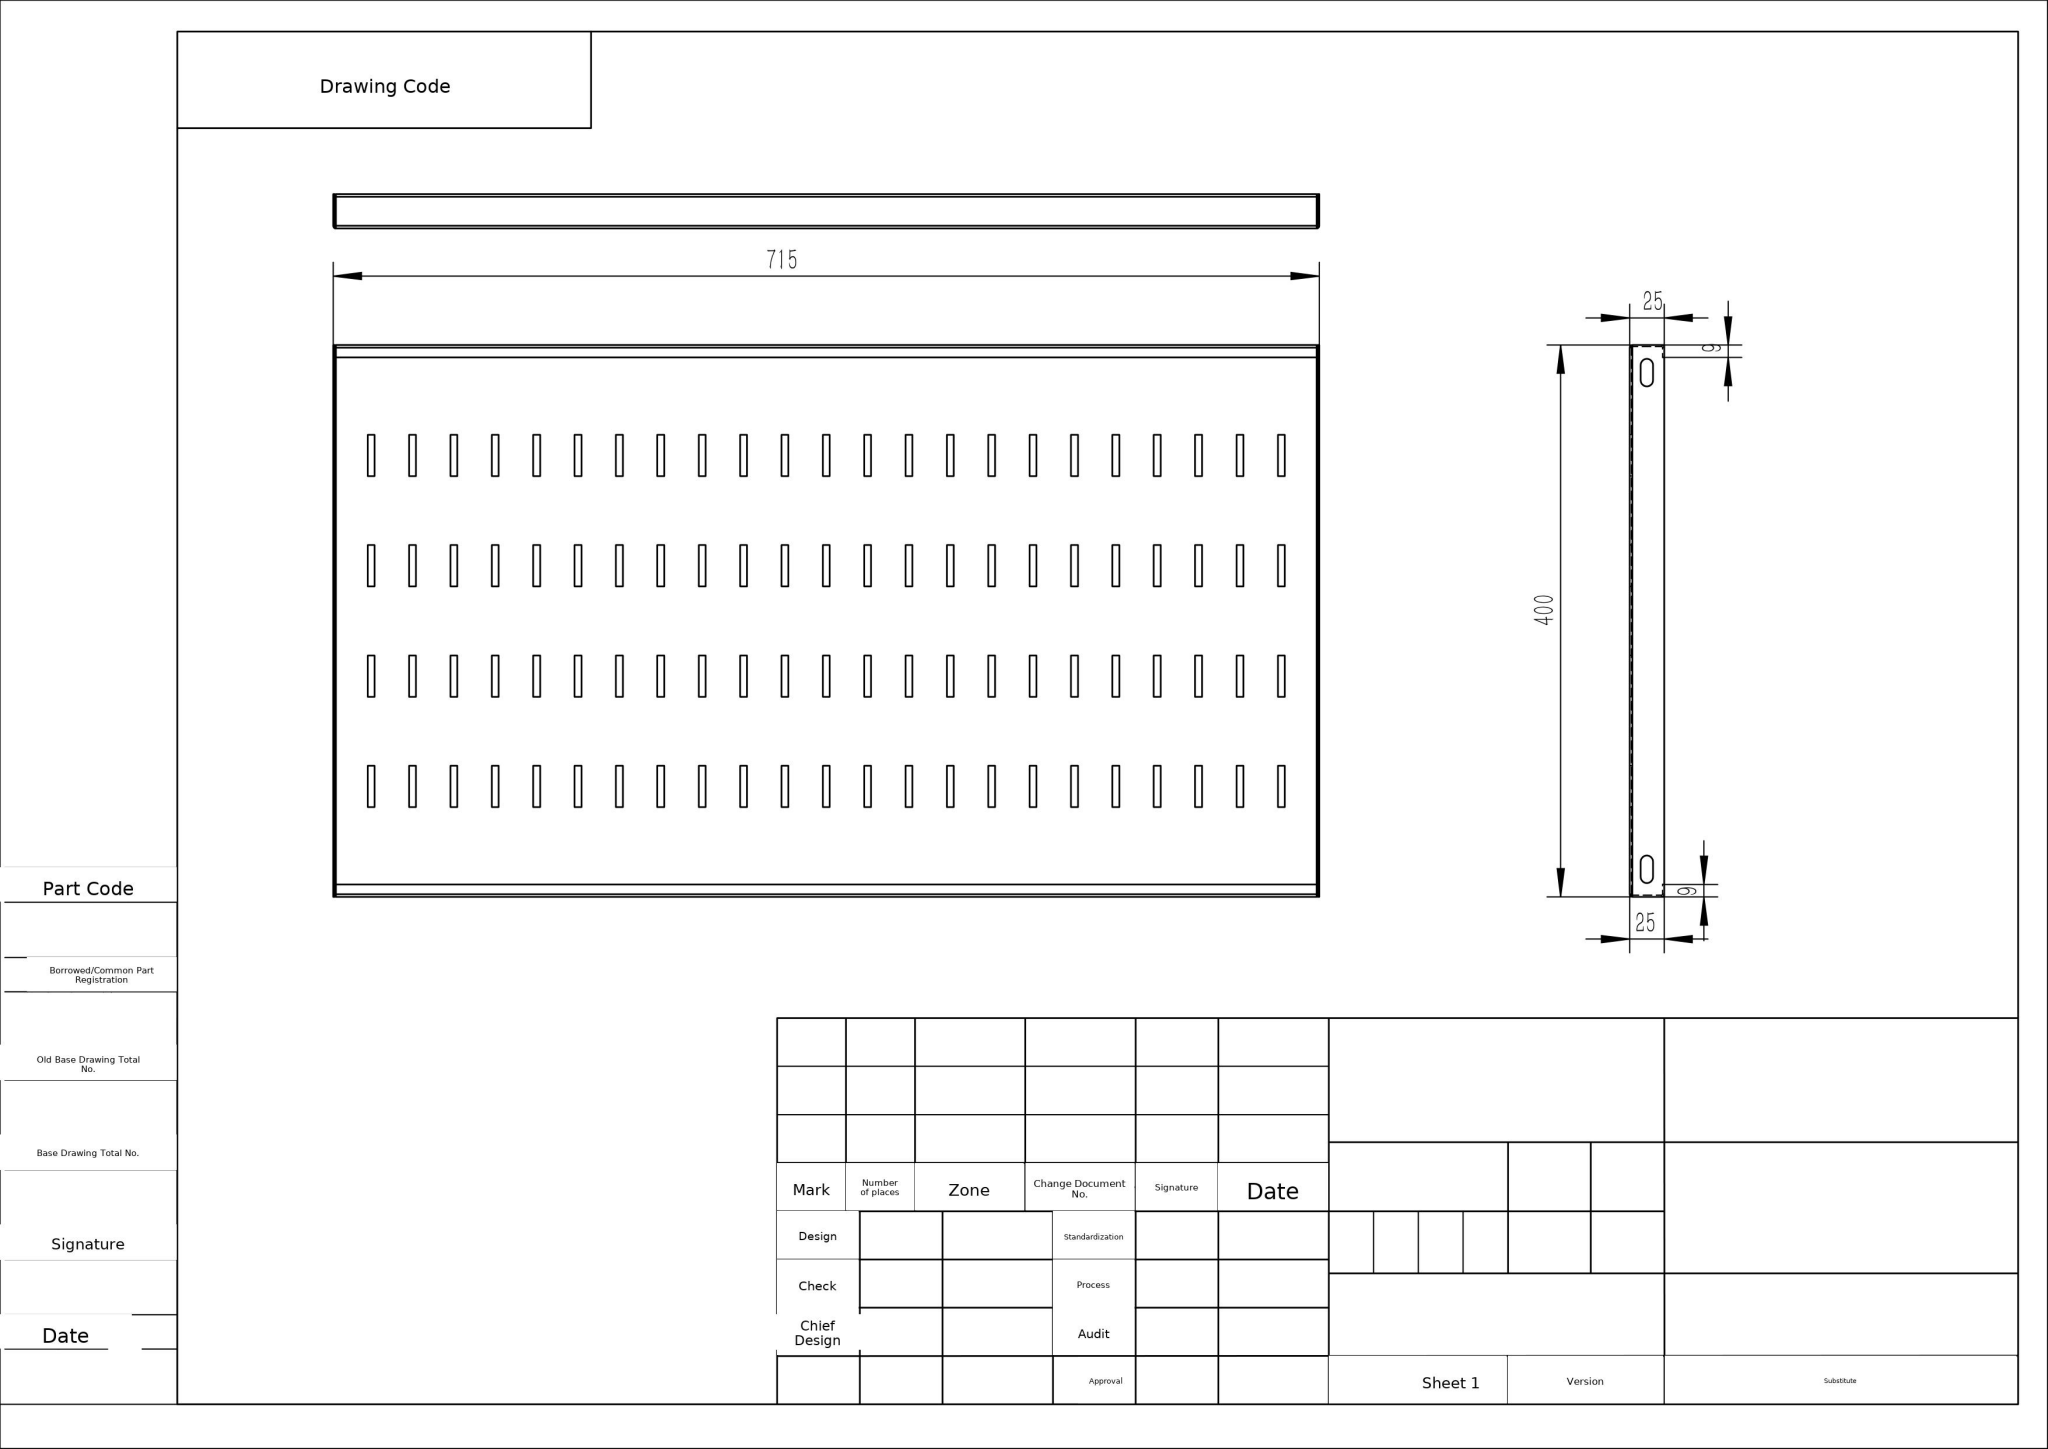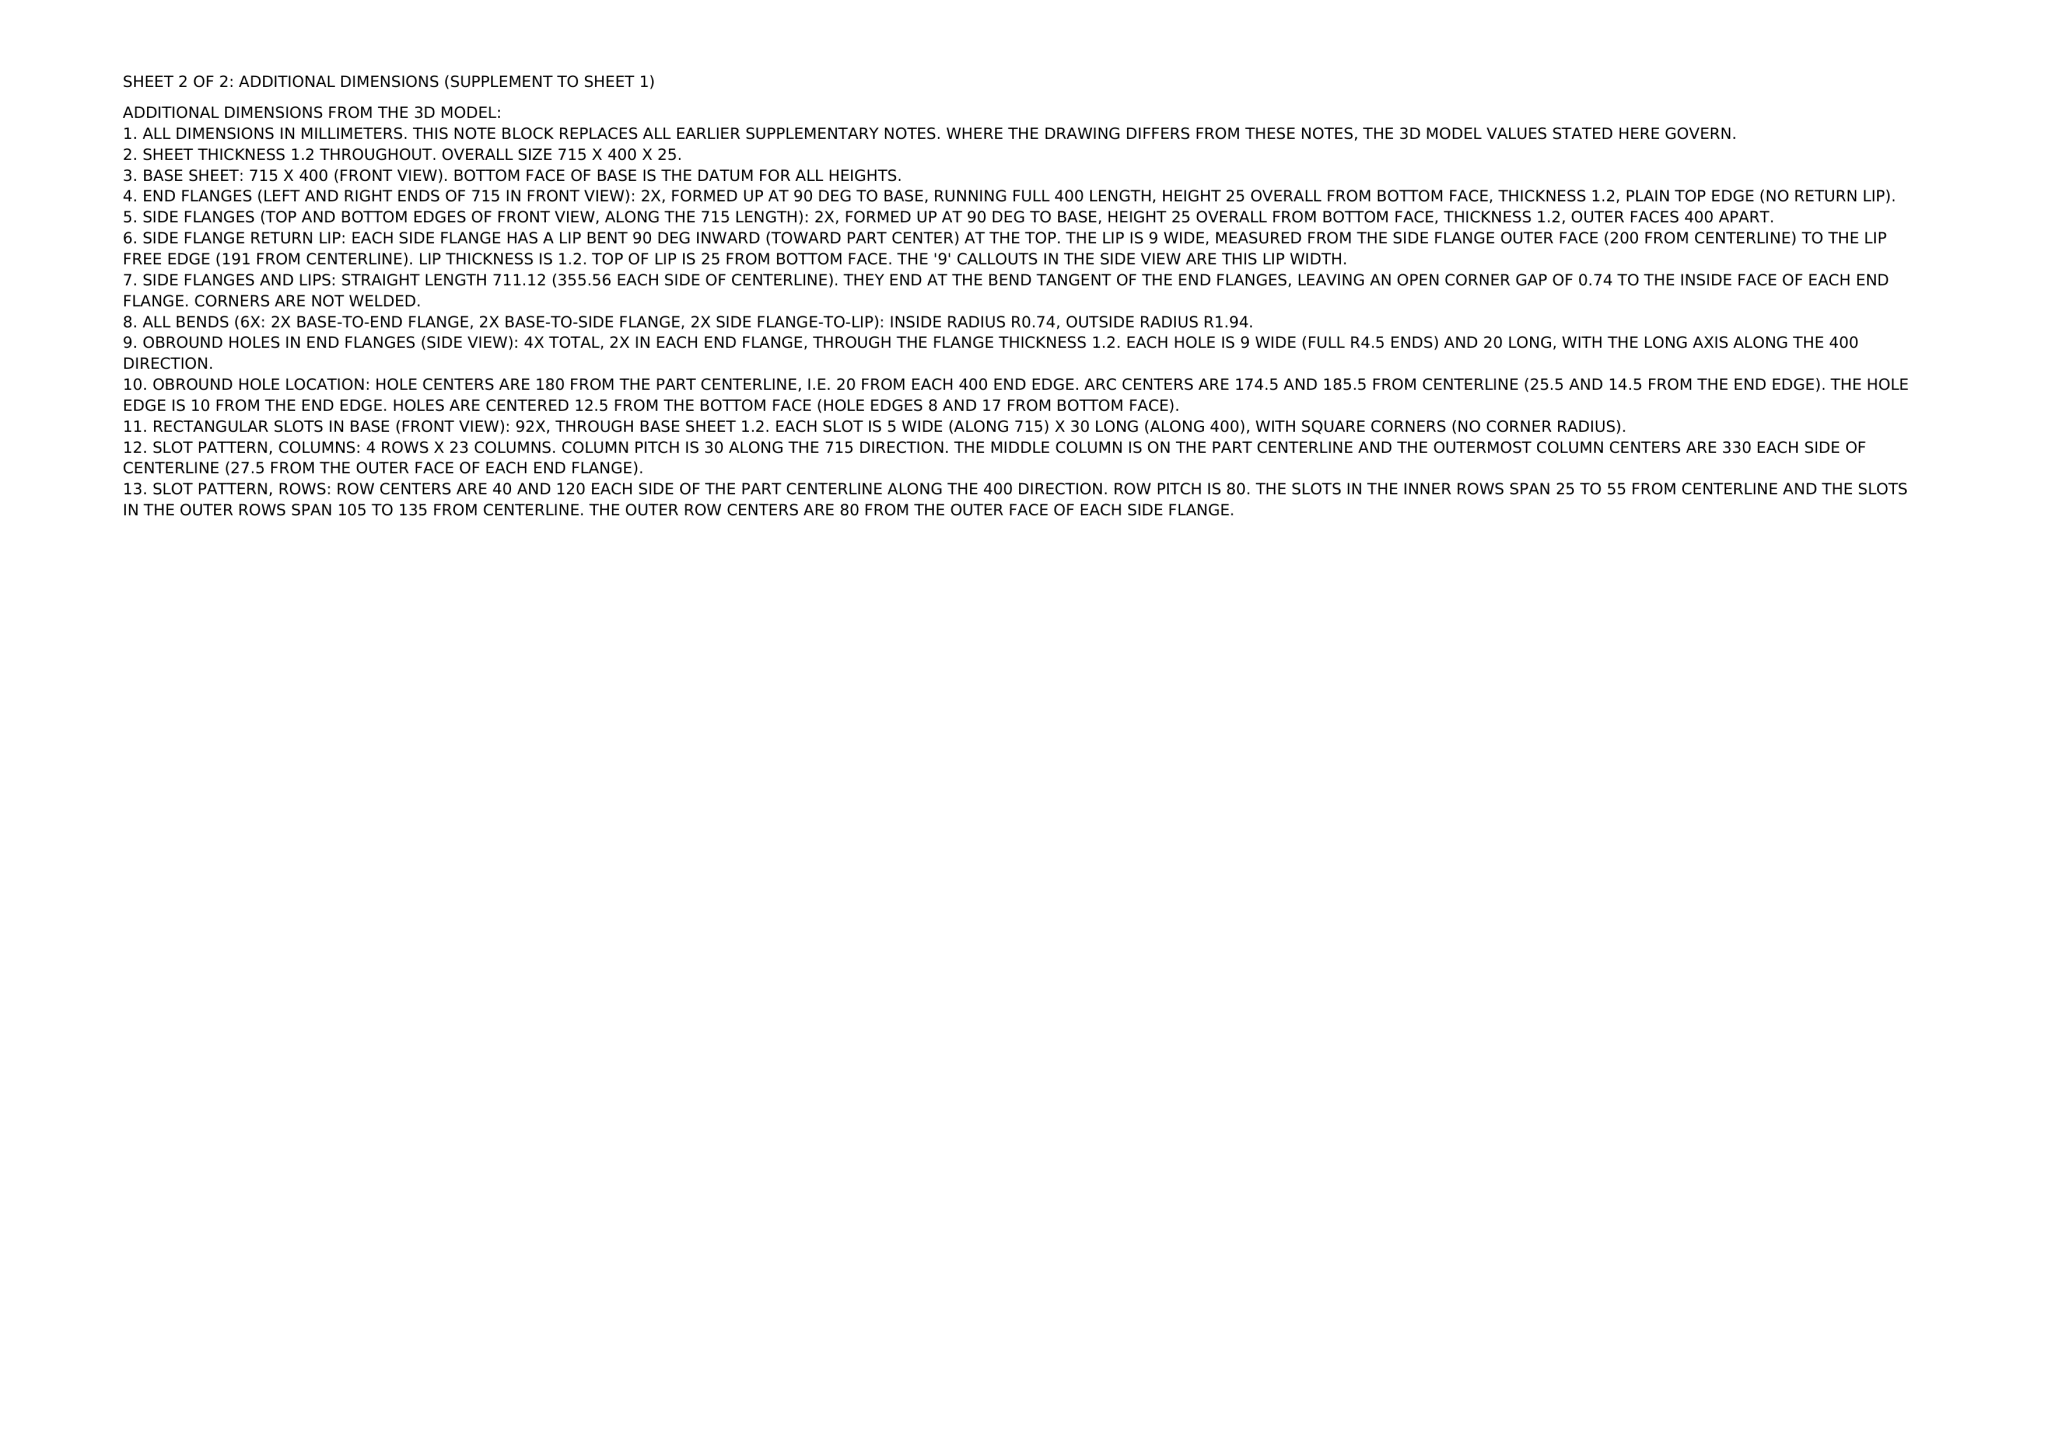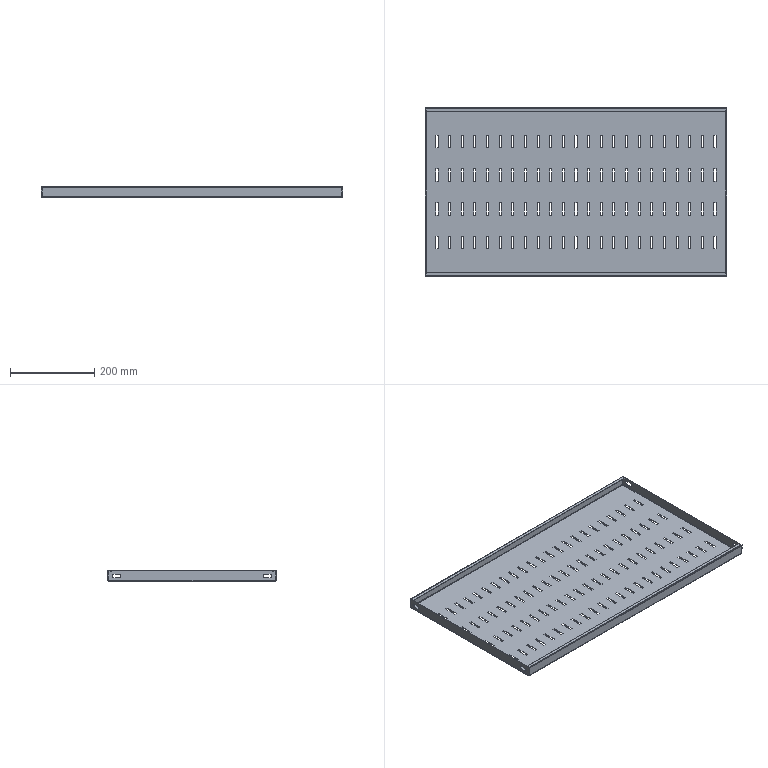Part | NX | mm | 1 solid | 438 faces | box 715 x 400 x 25 mm | volume 400121 mm3 | plane 414 | cylinder 20 | spline 4 | commonest cylinder face diameters 9 x8 3.873 x6 1.473 x6